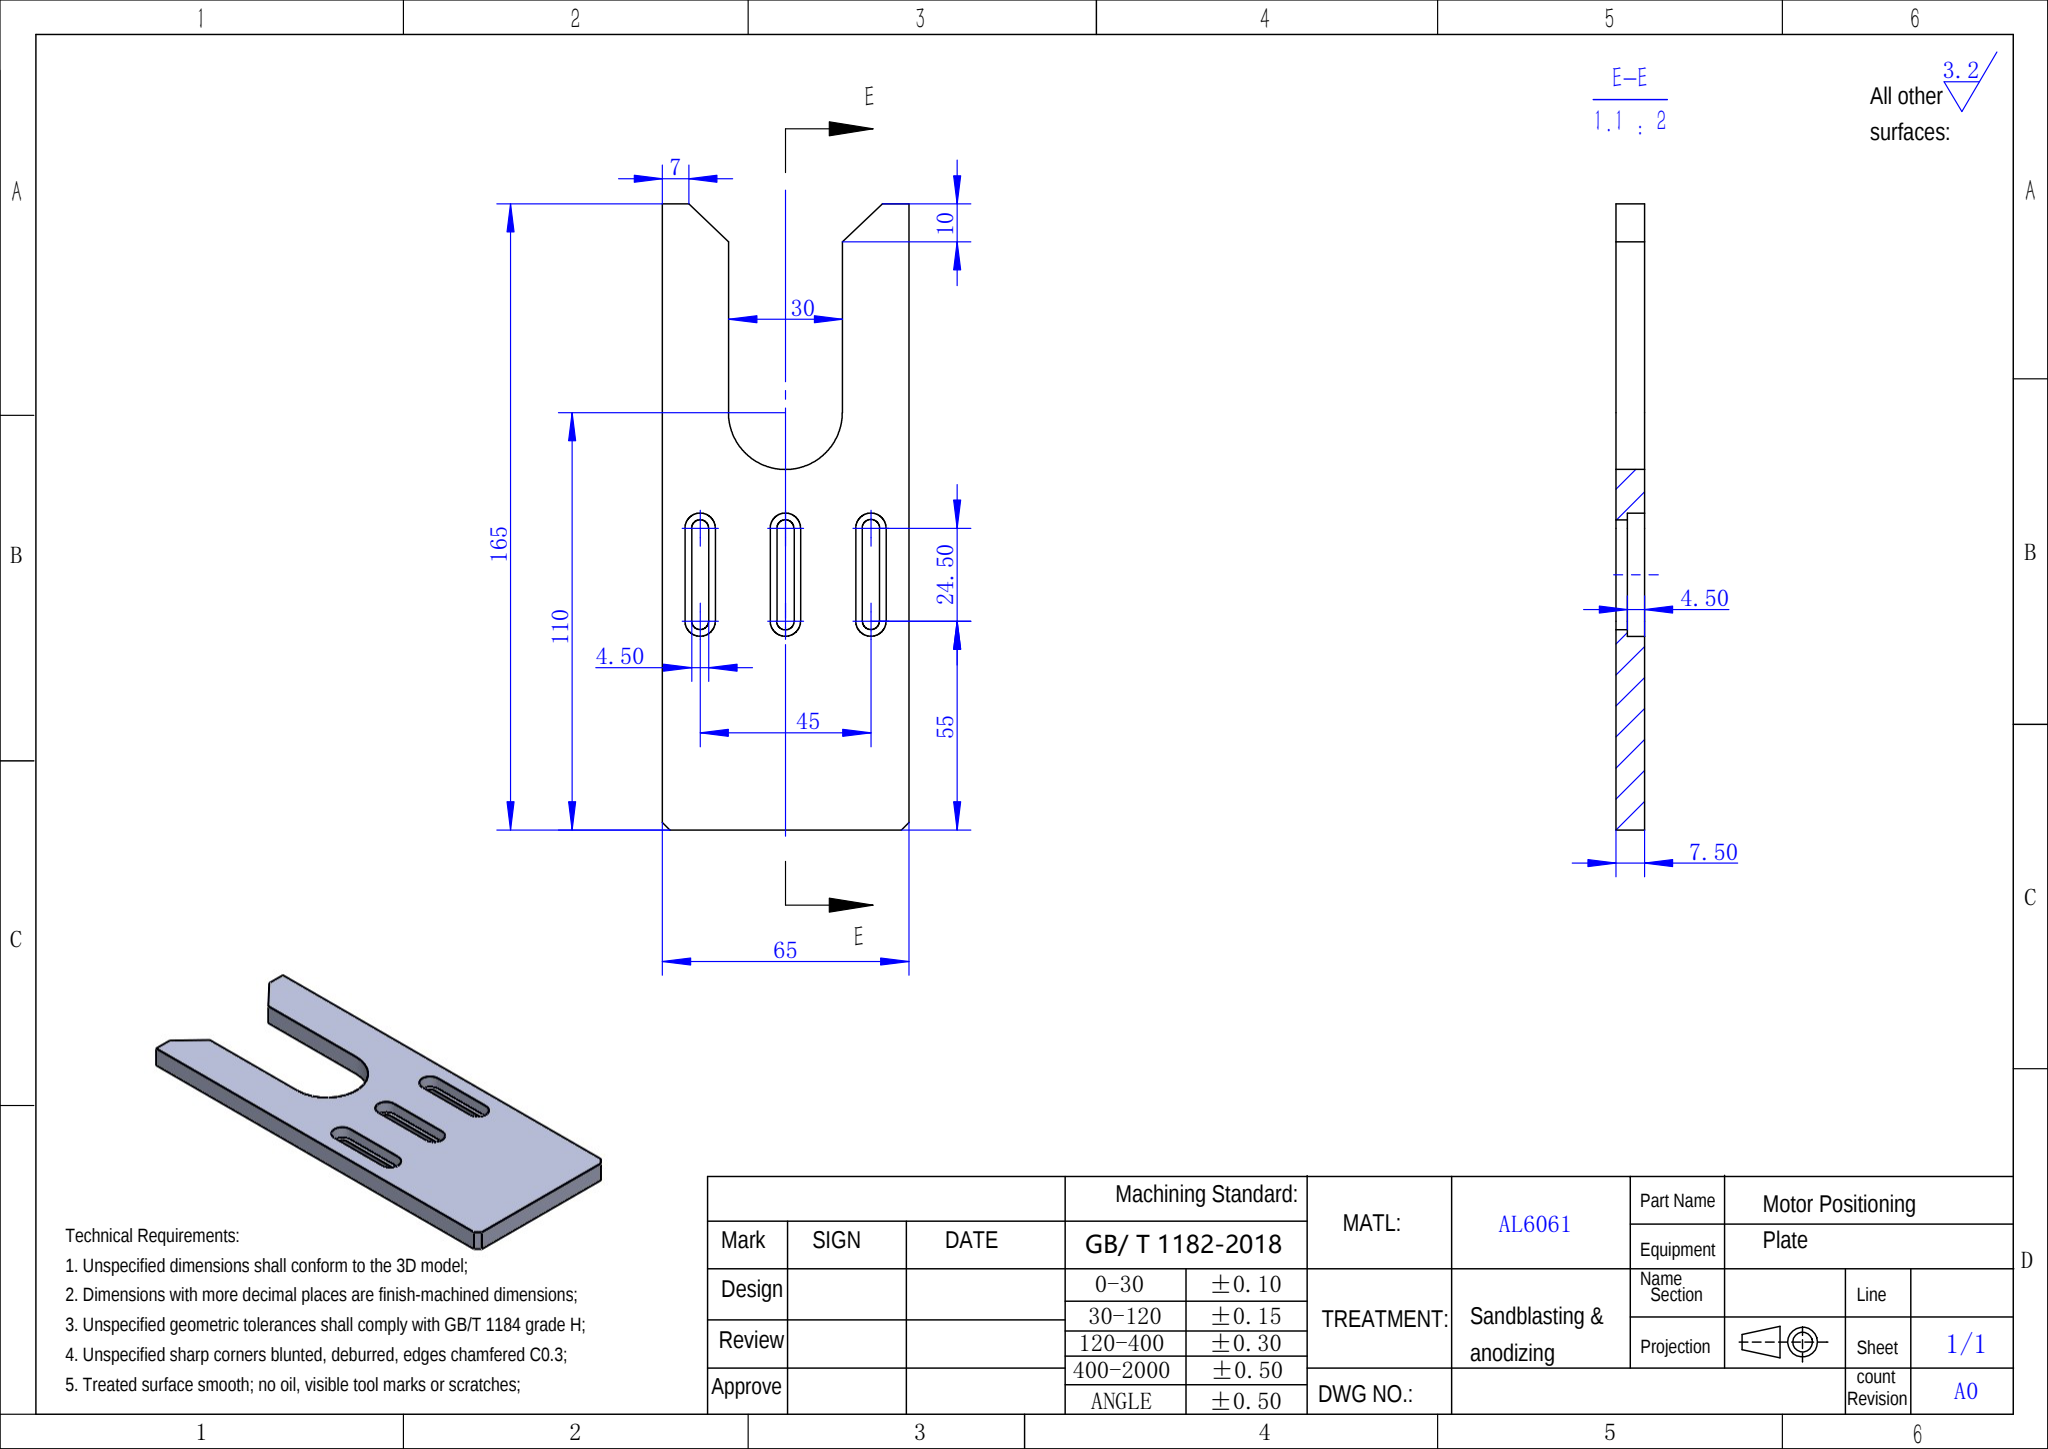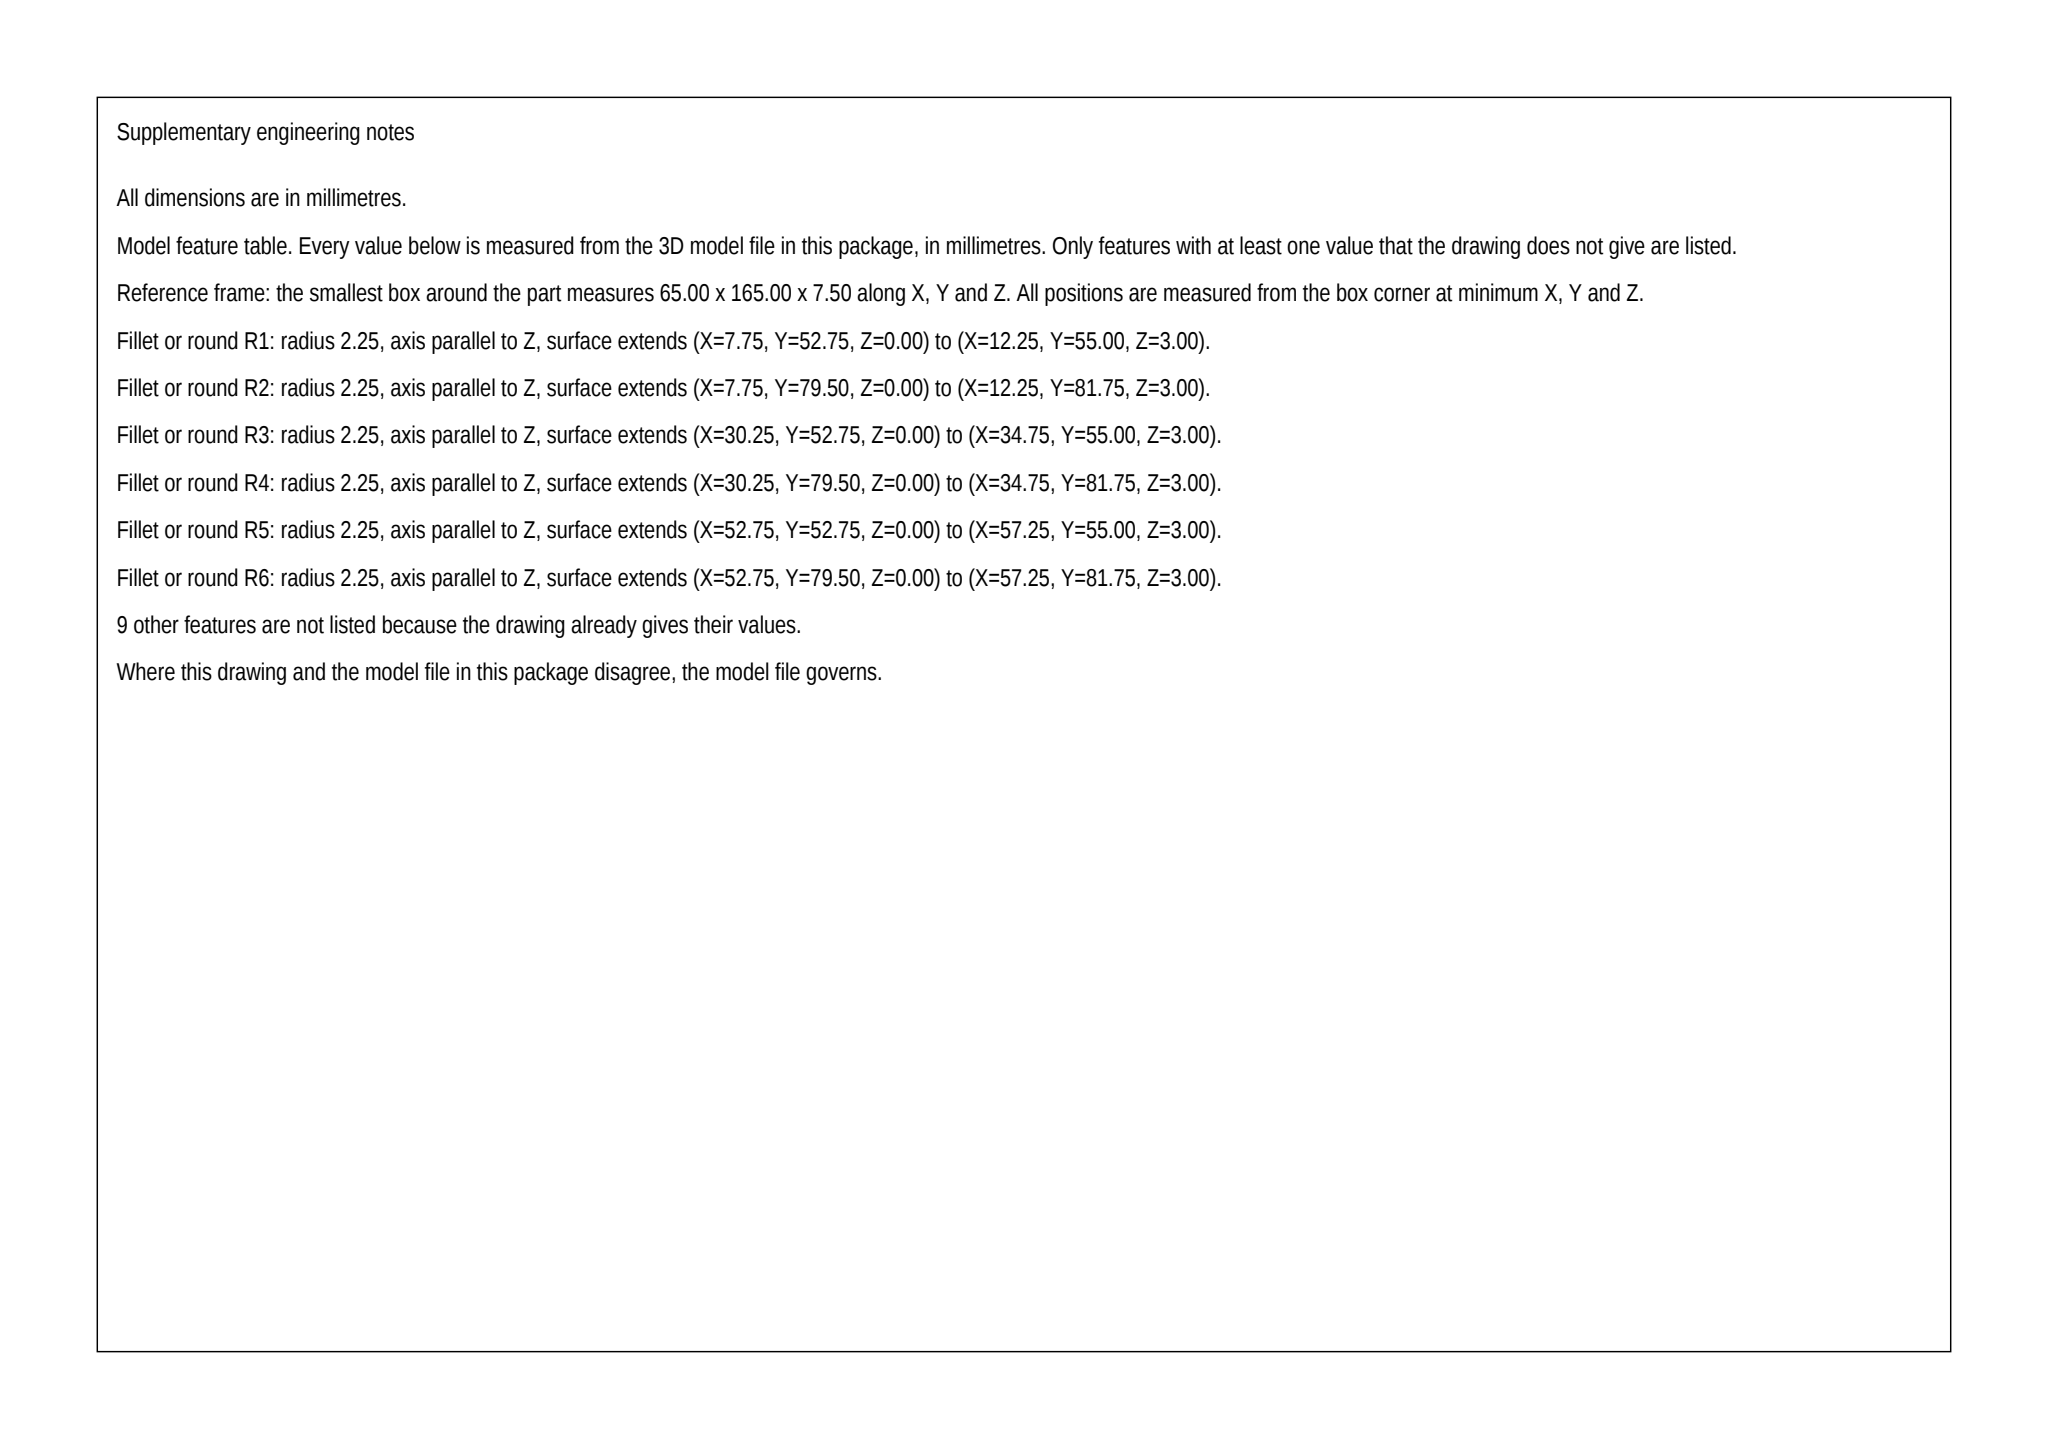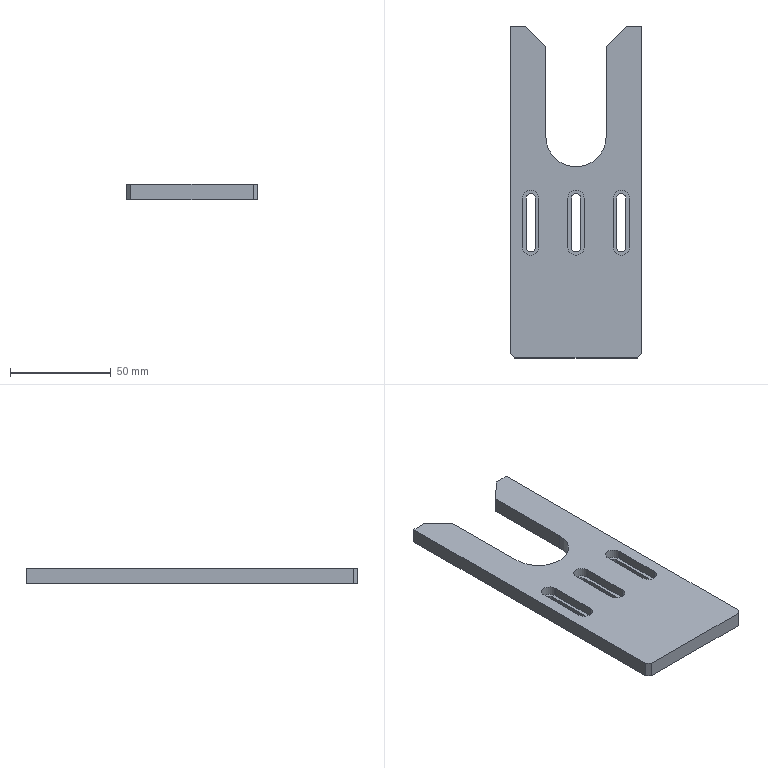Part | SolidWorks | mm | material AL6061 | 1 solid | 41 faces | box 65 x 165 x 7.5 mm | volume 60134 mm3 | plane 28 | cylinder 13 | commonest cylinder face diameters 4.5 x6 8 x6 30 x1
build123d program:
from build123d import *

# Parameters (mm, degrees)
BOSS_EXTRUDE1_DEPTH = 7.5
CUT_EXTRUDE1_DEPTH  = 169.337
CUT_EXTRUDE2_DEPTH  = 4.5
CHAMFER1_SIZE       = 2


with BuildPart() as part:
    # Sketch1 → Boss-Extrude1 (new body)
    with BuildSketch(Plane.XY):
        with BuildLine():
            Line((-32.5, 0), (32.5, 0))
            Line((32.5, 0), (32.5, 165))
            Line((32.5, 165), (25.5, 165))
            Line((25.5, 165), (15, 155))
            Line((15, 155), (15, 110))
            ThreePointArc((15, 110), (0, 95), (-15, 110))
            Line((-15, 110), (-15, 155))
            Line((-15, 155), (-25.5, 165))
            Line((-25.5, 165), (-32.5, 165))
            Line((-32.5, 165), (-32.5, 0))
        make_face()
    extrude(amount=BOSS_EXTRUDE1_DEPTH)

    # Sketch2 → Cut-Extrude1 (cut, through all)
    with BuildSketch(Plane.XY.offset(7.5)):
        with BuildLine():
            Line((2.25, 79.5), (2.25, 55))
            ThreePointArc((2.25, 55), (0, 52.75), (-2.25, 55))
            Line((-2.25, 55), (-2.25, 79.5))
            ThreePointArc((-2.25, 79.5), (0, 81.75), (2.25, 79.5))
        make_face()
        with BuildLine():
            Line((24.75, 79.5), (24.75, 55))
            ThreePointArc((24.75, 55), (22.5, 52.75), (20.25, 55))
            Line((20.25, 55), (20.25, 79.5))
            ThreePointArc((20.25, 79.5), (22.5, 81.75), (24.75, 79.5))
        make_face()
        with BuildLine():
            Line((-24.75, 79.5), (-24.75, 55))
            ThreePointArc((-24.75, 55), (-22.5, 52.75), (-20.25, 55))
            Line((-20.25, 55), (-20.25, 79.5))
            ThreePointArc((-20.25, 79.5), (-22.5, 81.75), (-24.75, 79.5))
        make_face()
    extrude(amount=-CUT_EXTRUDE1_DEPTH, mode=Mode.SUBTRACT)

    # Sketch3 → Cut-Extrude2 (cut)
    with BuildSketch(Plane.XY.offset(7.5)):
        with BuildLine():
            Line((-18.5, 55), (-18.5, 79.5))
            ThreePointArc((-18.5, 79.5), (-22.5, 83.5), (-26.5, 79.5))
            Line((-26.5, 79.5), (-26.5, 55))
            ThreePointArc((-26.5, 55), (-22.5, 51), (-18.5, 55))
        make_face()
        with BuildLine():
            Line((4, 55), (4, 79.5))
            ThreePointArc((4, 79.5), (0, 83.5), (-4, 79.5))
            Line((-4, 79.5), (-4, 55))
            ThreePointArc((-4, 55), (0, 51), (4, 55))
        make_face()
        with BuildLine():
            Line((18.5, 79.5), (18.5, 55))
            ThreePointArc((18.5, 55), (22.5, 51), (26.5, 55))
            Line((26.5, 55), (26.5, 79.5))
            ThreePointArc((26.5, 79.5), (22.5, 83.5), (18.5, 79.5))
        make_face()
    extrude(amount=-CUT_EXTRUDE2_DEPTH, mode=Mode.SUBTRACT)

    # Chamfer1
    chamfer1_edges = [part.edges().sort_by_distance(p)[0] for p in [
        (32.5, 0, 3.75),
        (-32.5, 0, 3.75),
    ]]
    chamfer(chamfer1_edges, length=CHAMFER1_SIZE)


solid = part.part